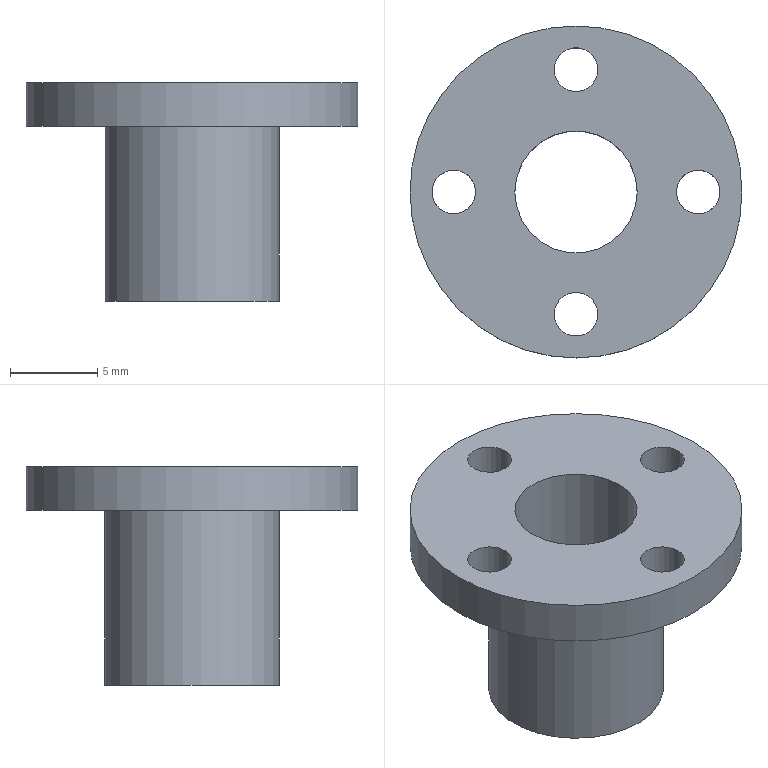Component | NX | EXT_CYLINDER_END_COVER | 1 solid | 10 faces | volume 964 mm3 | cylinder 7 | plane 3 | commonest cylinder face diameters 2.5 x4 10 x1 19 x1 7 x1